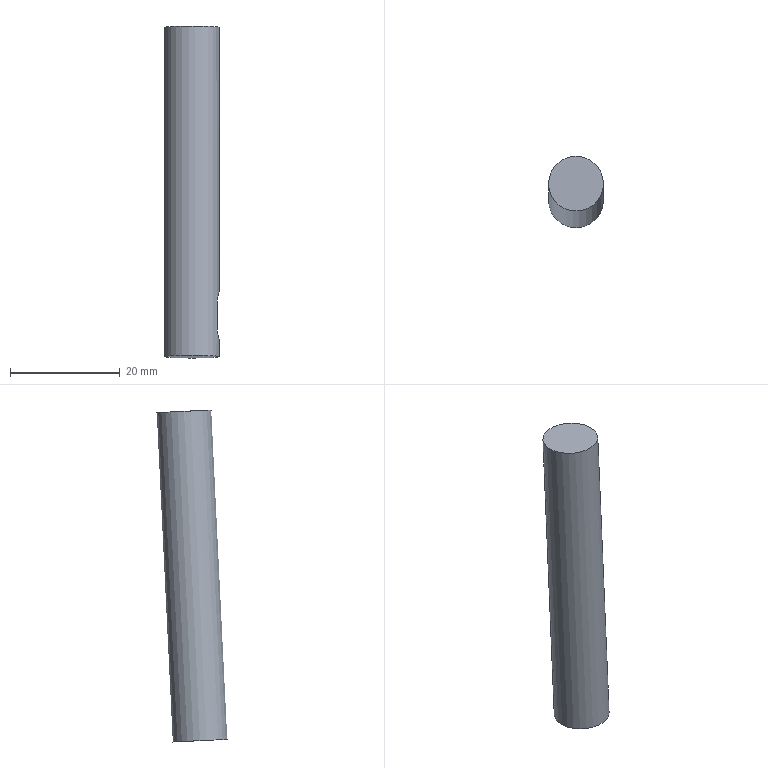Component | NX | CCJ-022 | 1 solid | 8 faces | box 10 x 12.91 x 60.42 mm | volume 4658 mm3 | plane 5 | cylinder 3 | commonest cylinder face diameters 4 x2 10 x1
STEP:
#1=CARTESIAN_POINT('',(0.,0.,0.));
#2=DIRECTION('',(0.,0.,1.));
#3=DIRECTION('',(1.,0.,0.));
#4=AXIS2_PLACEMENT_3D('',#1,#2,#3);
#5=CARTESIAN_POINT('',(30.,442.597,164.469));
#6=VERTEX_POINT('',#5);
#7=CARTESIAN_POINT('',(25.,442.597,164.469));
#8=DIRECTION('',(0.,0.04861,0.9988));
#9=DIRECTION('',(1.,0.,0.));
#10=AXIS2_PLACEMENT_3D('',#7,#8,#9);
#11=CIRCLE('',#10,5.);
#12=CARTESIAN_POINT('',(25.,445.514,224.398));
#13=DIRECTION('',(0.,-0.04861,-0.9988));
#14=DIRECTION('',(-1.,0.,0.));
#15=AXIS2_PLACEMENT_3D('',#12,#13,#14);
#16=CYLINDRICAL_SURFACE('',#15,5.);
#17=CARTESIAN_POINT('',(9.425,60.));
#18=DIRECTION('',(-1.,0.));
#19=VECTOR('',#18,1.);
#20=LINE('',#17,#19);
#21=(GEOMETRIC_REPRESENTATION_CONTEXT(2)PARAMETRIC_REPRESENTATION_CONTEXT()REPRESENTATION_CONTEXT('',''));
#22=DEFINITIONAL_REPRESENTATION('',(#20),#21);
#23=PCURVE('',#16,#22);
#24=CARTESIAN_POINT('',(25.,442.597,164.469));
#25=DIRECTION('',(0.,0.04861,0.9988));
#26=DIRECTION('',(1.,0.,0.));
#27=AXIS2_PLACEMENT_3D('',#24,#25,#26);
#28=PLANE('',#27);
#29=CARTESIAN_POINT('',(0.,0.));
#30=DIRECTION('',(1.,0.));
#31=AXIS2_PLACEMENT_2D('',#29,#30);
#32=CIRCLE('',#31,5.);
#33=(GEOMETRIC_REPRESENTATION_CONTEXT(2)PARAMETRIC_REPRESENTATION_CONTEXT()REPRESENTATION_CONTEXT('',''));
#34=DEFINITIONAL_REPRESENTATION('',(#32),#33);
#35=PCURVE('',#28,#34);
#36=SURFACE_CURVE('',#11,(#23,#35),.PCURVE_S1.);
#37=EDGE_CURVE('',#6,#6,#36,.T.);
#38=ORIENTED_EDGE('',*,*,#37,.T.);
#39=CARTESIAN_POINT('',(30.,442.743,167.466));
#40=VERTEX_POINT('',#39);
#41=CARTESIAN_POINT('',(30.,442.743,167.466));
#42=CARTESIAN_POINT('',(30.,442.597,164.469));
#43=B_SPLINE_CURVE_WITH_KNOTS('',1,(#41,#42),.UNSPECIFIED.,.F.,.F.,(2,2),(57.,60.),.PIECEWISE_BEZIER_KNOTS.);
#44=CARTESIAN_POINT('',(3.142,0.));
#45=DIRECTION('',(0.,1.));
#46=VECTOR('',#45,1.);
#47=LINE('',#44,#46);
#48=(GEOMETRIC_REPRESENTATION_CONTEXT(2)PARAMETRIC_REPRESENTATION_CONTEXT()REPRESENTATION_CONTEXT('',''));
#49=DEFINITIONAL_REPRESENTATION('',(#47),#48);
#50=PCURVE('',#16,#49);
#51=CARTESIAN_POINT('',(9.425,0.));
#52=DIRECTION('',(0.,1.));
#53=VECTOR('',#52,1.);
#54=LINE('',#51,#53);
#55=(GEOMETRIC_REPRESENTATION_CONTEXT(2)PARAMETRIC_REPRESENTATION_CONTEXT()REPRESENTATION_CONTEXT('',''));
#56=DEFINITIONAL_REPRESENTATION('',(#54),#55);
#57=PCURVE('',#16,#56);
#58=SEAM_CURVE('',#43,(#50,#57),.PCURVE_S1.);
#59=EDGE_CURVE('',#40,#6,#58,.T.);
#60=ORIENTED_EDGE('',*,*,#59,.F.);
#61=CARTESIAN_POINT('',(29.583,440.843,169.56));
#62=VERTEX_POINT('',#61);
#63=CARTESIAN_POINT('',(29.583,440.843,169.56));
#64=CARTESIAN_POINT('',(29.583,440.832,169.347));
#65=CARTESIAN_POINT('',(29.598,440.857,169.129));
#66=CARTESIAN_POINT('',(29.626,440.914,168.925));
#67=CARTESIAN_POINT('',(29.653,440.971,168.721));
#68=CARTESIAN_POINT('',(29.692,441.061,168.526));
#69=CARTESIAN_POINT('',(29.735,441.177,168.352));
#70=CARTESIAN_POINT('',(29.779,441.299,168.169));
#71=CARTESIAN_POINT('',(29.828,441.453,168.005));
#72=CARTESIAN_POINT('',(29.87,441.629,167.872));
#73=CARTESIAN_POINT('',(29.914,441.811,167.733));
#74=CARTESIAN_POINT('',(29.952,442.021,167.624));
#75=CARTESIAN_POINT('',(29.975,442.243,167.554));
#76=CARTESIAN_POINT('',(29.996,442.453,167.489));
#77=CARTESIAN_POINT('',(30.004,442.679,167.457));
#78=CARTESIAN_POINT('',(29.998,442.901,167.464));
#79=CARTESIAN_POINT('',(29.991,443.11,167.47));
#80=CARTESIAN_POINT('',(29.971,443.32,167.51));
#81=CARTESIAN_POINT('',(29.941,443.515,167.58));
#82=CARTESIAN_POINT('',(29.911,443.713,167.651));
#83=CARTESIAN_POINT('',(29.871,443.9,167.754));
#84=CARTESIAN_POINT('',(29.828,444.065,167.882));
#85=CARTESIAN_POINT('',(29.783,444.24,168.018));
#86=CARTESIAN_POINT('',(29.734,444.395,168.185));
#87=CARTESIAN_POINT('',(29.692,444.516,168.371));
#88=CARTESIAN_POINT('',(29.65,444.641,168.563));
#89=CARTESIAN_POINT('',(29.615,444.735,168.781));
#90=CARTESIAN_POINT('',(29.597,444.788,169.007));
#91=CARTESIAN_POINT('',(29.587,444.815,169.124));
#92=CARTESIAN_POINT('',(29.583,444.832,169.245));
#93=CARTESIAN_POINT('',(29.583,444.838,169.366));
#94=B_SPLINE_CURVE_WITH_KNOTS('',3,(#63,#64,#65,#66,#67,#68,#69,#70,#71,#72,#73,#74,#75,#76,#77,#78,#79,#80,#81,#82,#83,#84,#85,#86,#87,#88,#89,#90,#91,#92,#93),.UNSPECIFIED.,.F.,.F.,(4,3,3,3,3,3,3,3,3,3,4),(0.,0.1015,0.2026,0.309,0.4198,0.5251,0.6244,0.7251,0.8326,0.9432,1.),.UNSPECIFIED.);
#95=CARTESIAN_POINT('',(3.553,55.));
#96=CARTESIAN_POINT('',(3.553,55.048));
#97=CARTESIAN_POINT('',(3.552,55.144));
#98=CARTESIAN_POINT('',(3.549,55.287));
#99=CARTESIAN_POINT('',(3.543,55.43));
#100=CARTESIAN_POINT('',(3.536,55.569));
#101=CARTESIAN_POINT('',(3.526,55.704));
#102=CARTESIAN_POINT('',(3.514,55.836));
#103=CARTESIAN_POINT('',(3.5,55.963));
#104=CARTESIAN_POINT('',(3.485,56.085));
#105=CARTESIAN_POINT('',(3.468,56.201));
#106=CARTESIAN_POINT('',(3.449,56.311));
#107=CARTESIAN_POINT('',(3.429,56.415));
#108=CARTESIAN_POINT('',(3.407,56.511));
#109=CARTESIAN_POINT('',(3.384,56.6));
#110=CARTESIAN_POINT('',(3.361,56.681));
#111=CARTESIAN_POINT('',(3.336,56.754));
#112=CARTESIAN_POINT('',(3.31,56.818));
#113=CARTESIAN_POINT('',(3.283,56.873));
#114=CARTESIAN_POINT('',(3.256,56.919));
#115=CARTESIAN_POINT('',(3.228,56.955));
#116=CARTESIAN_POINT('',(3.2,56.98));
#117=CARTESIAN_POINT('',(3.171,56.996));
#118=CARTESIAN_POINT('',(3.142,57.002));
#119=CARTESIAN_POINT('',(3.113,56.997));
#120=CARTESIAN_POINT('',(3.084,56.981));
#121=CARTESIAN_POINT('',(3.056,56.955));
#122=CARTESIAN_POINT('',(3.028,56.92));
#123=CARTESIAN_POINT('',(3.,56.874));
#124=CARTESIAN_POINT('',(2.974,56.819));
#125=CARTESIAN_POINT('',(2.948,56.755));
#126=CARTESIAN_POINT('',(2.923,56.682));
#127=CARTESIAN_POINT('',(2.899,56.601));
#128=CARTESIAN_POINT('',(2.876,56.512));
#129=CARTESIAN_POINT('',(2.855,56.416));
#130=CARTESIAN_POINT('',(2.835,56.312));
#131=CARTESIAN_POINT('',(2.816,56.202));
#132=CARTESIAN_POINT('',(2.799,56.086));
#133=CARTESIAN_POINT('',(2.783,55.965));
#134=CARTESIAN_POINT('',(2.77,55.838));
#135=CARTESIAN_POINT('',(2.758,55.706));
#136=CARTESIAN_POINT('',(2.748,55.57));
#137=CARTESIAN_POINT('',(2.74,55.432));
#138=CARTESIAN_POINT('',(2.734,55.29));
#139=CARTESIAN_POINT('',(2.731,55.145));
#140=CARTESIAN_POINT('',(2.73,55.048));
#141=CARTESIAN_POINT('',(2.73,55.));
#142=B_SPLINE_CURVE_WITH_KNOTS('',3,(#95,#96,#97,#98,#99,#100,#101,#102,#103,#104,#105,#106,#107,#108,#109,#110,#111,#112,#113,#114,#115,#116,#117,#118,#119,#120,#121,#122,#123,#124,#125,#126,#127,#128,#129,#130,#131,#132,#133,#134,#135,#136,#137,#138,#139,#140,#141),.UNSPECIFIED.,.F.,.F.,(4,1,1,1,1,1,1,1,1,1,1,1,1,1,1,1,1,1,1,1,1,1,1,1,1,1,1,1,1,1,1,1,1,1,1,1,1,1,1,1,1,1,1,1,4),(0.,0.02273,0.04545,0.06818,0.09091,0.1136,0.1364,0.1591,0.1818,0.2045,0.2273,0.25,0.2727,0.2955,0.3182,0.3409,0.3636,0.3864,0.4091,0.4318,0.4545,0.4773,0.5,0.5227,0.5455,0.5682,0.5909,0.6136,0.6364,0.6591,0.6818,0.7045,0.7273,0.75,0.7727,0.7955,0.8182,0.8409,0.8636,0.8864,0.9091,0.9318,0.9545,0.9773,1.),.QUASI_UNIFORM_KNOTS.);
#143=(GEOMETRIC_REPRESENTATION_CONTEXT(2)PARAMETRIC_REPRESENTATION_CONTEXT()REPRESENTATION_CONTEXT('',''));
#144=DEFINITIONAL_REPRESENTATION('',(#142),#143);
#145=PCURVE('',#16,#144);
#146=CARTESIAN_POINT('',(40.,442.84,169.463));
#147=DIRECTION('',(-1.,0.,0.));
#148=DIRECTION('',(0.,0.04861,0.9988));
#149=AXIS2_PLACEMENT_3D('',#146,#147,#148);
#150=CYLINDRICAL_SURFACE('',#149,2.);
#151=CARTESIAN_POINT('',(4.712,10.417));
#152=CARTESIAN_POINT('',(3.142,10.));
#153=B_SPLINE_CURVE_WITH_KNOTS('',1,(#151,#152),.UNSPECIFIED.,.F.,.F.,(2,2),(0.,0.5002),.PIECEWISE_BEZIER_KNOTS.);
#154=(GEOMETRIC_REPRESENTATION_CONTEXT(2)PARAMETRIC_REPRESENTATION_CONTEXT()REPRESENTATION_CONTEXT('',''));
#155=DEFINITIONAL_REPRESENTATION('',(#153),#154);
#156=PCURVE('',#150,#155);
#157=SURFACE_CURVE('',#94,(#145,#156),.PCURVE_S1.);
#158=EDGE_CURVE('',#62,#40,#157,.T.);
#159=ORIENTED_EDGE('',*,*,#158,.F.);
#160=CARTESIAN_POINT('',(29.583,441.086,174.554));
#161=VERTEX_POINT('',#160);
#162=CARTESIAN_POINT('',(29.583,443.516,224.495));
#163=DIRECTION('',(0.,-0.04861,-0.9988));
#164=VECTOR('',#163,1.);
#165=LINE('',#162,#164);
#166=CARTESIAN_POINT('',(3.553,0.));
#167=DIRECTION('',(-0.,1.));
#168=VECTOR('',#167,1.);
#169=LINE('',#166,#168);
#170=(GEOMETRIC_REPRESENTATION_CONTEXT(2)PARAMETRIC_REPRESENTATION_CONTEXT()REPRESENTATION_CONTEXT('',''));
#171=DEFINITIONAL_REPRESENTATION('',(#169),#170);
#172=PCURVE('',#16,#171);
#173=CARTESIAN_POINT('',(40.,441.086,174.554));
#174=DIRECTION('',(0.,0.9988,-0.04861));
#175=DIRECTION('',(0.,0.04861,0.9988));
#176=AXIS2_PLACEMENT_3D('',#173,#174,#175);
#177=PLANE('',#176);
#178=CARTESIAN_POINT('',(50.,-10.417));
#179=DIRECTION('',(-1.,0.));
#180=VECTOR('',#179,1.);
#181=LINE('',#178,#180);
#182=(GEOMETRIC_REPRESENTATION_CONTEXT(2)PARAMETRIC_REPRESENTATION_CONTEXT()REPRESENTATION_CONTEXT('',''));
#183=DEFINITIONAL_REPRESENTATION('',(#181),#182);
#184=PCURVE('',#177,#183);
#185=SURFACE_CURVE('',#165,(#172,#184),.PCURVE_S1.);
#186=EDGE_CURVE('',#161,#62,#185,.T.);
#187=ORIENTED_EDGE('',*,*,#186,.F.);
#188=CARTESIAN_POINT('',(30.,443.181,176.455));
#189=VERTEX_POINT('',#188);
#190=CARTESIAN_POINT('',(29.583,445.081,174.36));
#191=CARTESIAN_POINT('',(29.583,445.091,174.573));
#192=CARTESIAN_POINT('',(29.598,445.067,174.791));
#193=CARTESIAN_POINT('',(29.626,445.01,174.995));
#194=CARTESIAN_POINT('',(29.653,444.953,175.199));
#195=CARTESIAN_POINT('',(29.692,444.862,175.394));
#196=CARTESIAN_POINT('',(29.735,444.746,175.568));
#197=CARTESIAN_POINT('',(29.779,444.624,175.751));
#198=CARTESIAN_POINT('',(29.828,444.47,175.915));
#199=CARTESIAN_POINT('',(29.87,444.295,176.048));
#200=CARTESIAN_POINT('',(29.914,444.113,176.187));
#201=CARTESIAN_POINT('',(29.952,443.902,176.296));
#202=CARTESIAN_POINT('',(29.975,443.681,176.366));
#203=CARTESIAN_POINT('',(29.996,443.471,176.432));
#204=CARTESIAN_POINT('',(30.004,443.244,176.463));
#205=CARTESIAN_POINT('',(29.998,443.023,176.456));
#206=CARTESIAN_POINT('',(29.991,442.814,176.45));
#207=CARTESIAN_POINT('',(29.971,442.604,176.41));
#208=CARTESIAN_POINT('',(29.941,442.409,176.34));
#209=CARTESIAN_POINT('',(29.911,442.211,176.269));
#210=CARTESIAN_POINT('',(29.871,442.023,176.166));
#211=CARTESIAN_POINT('',(29.828,441.859,176.038));
#212=CARTESIAN_POINT('',(29.783,441.683,175.902));
#213=CARTESIAN_POINT('',(29.734,441.529,175.735));
#214=CARTESIAN_POINT('',(29.692,441.408,175.549));
#215=CARTESIAN_POINT('',(29.65,441.283,175.357));
#216=CARTESIAN_POINT('',(29.615,441.189,175.139));
#217=CARTESIAN_POINT('',(29.597,441.136,174.913));
#218=CARTESIAN_POINT('',(29.587,441.109,174.796));
#219=CARTESIAN_POINT('',(29.583,441.092,174.675));
#220=CARTESIAN_POINT('',(29.583,441.086,174.554));
#221=B_SPLINE_CURVE_WITH_KNOTS('',3,(#190,#191,#192,#193,#194,#195,#196,#197,#198,#199,#200,#201,#202,#203,#204,#205,#206,#207,#208,#209,#210,#211,#212,#213,#214,#215,#216,#217,#218,#219,#220),.UNSPECIFIED.,.F.,.F.,(4,3,3,3,3,3,3,3,3,3,4),(0.,0.1015,0.2026,0.309,0.4198,0.5251,0.6244,0.7251,0.8326,0.9432,1.),.UNSPECIFIED.);
#222=CARTESIAN_POINT('',(2.73,50.));
#223=CARTESIAN_POINT('',(2.73,49.952));
#224=CARTESIAN_POINT('',(2.731,49.856));
#225=CARTESIAN_POINT('',(2.734,49.713));
#226=CARTESIAN_POINT('',(2.74,49.57));
#227=CARTESIAN_POINT('',(2.748,49.431));
#228=CARTESIAN_POINT('',(2.757,49.296));
#229=CARTESIAN_POINT('',(2.769,49.164));
#230=CARTESIAN_POINT('',(2.783,49.037));
#231=CARTESIAN_POINT('',(2.799,48.915));
#232=CARTESIAN_POINT('',(2.816,48.799));
#233=CARTESIAN_POINT('',(2.834,48.689));
#234=CARTESIAN_POINT('',(2.855,48.585));
#235=CARTESIAN_POINT('',(2.876,48.489));
#236=CARTESIAN_POINT('',(2.899,48.4));
#237=CARTESIAN_POINT('',(2.923,48.319));
#238=CARTESIAN_POINT('',(2.947,48.246));
#239=CARTESIAN_POINT('',(2.973,48.182));
#240=CARTESIAN_POINT('',(3.,48.127));
#241=CARTESIAN_POINT('',(3.027,48.081));
#242=CARTESIAN_POINT('',(3.055,48.045));
#243=CARTESIAN_POINT('',(3.084,48.02));
#244=CARTESIAN_POINT('',(3.112,48.004));
#245=CARTESIAN_POINT('',(3.141,47.998));
#246=CARTESIAN_POINT('',(3.17,48.003));
#247=CARTESIAN_POINT('',(3.199,48.019));
#248=CARTESIAN_POINT('',(3.227,48.045));
#249=CARTESIAN_POINT('',(3.255,48.08));
#250=CARTESIAN_POINT('',(3.283,48.126));
#251=CARTESIAN_POINT('',(3.309,48.181));
#252=CARTESIAN_POINT('',(3.335,48.245));
#253=CARTESIAN_POINT('',(3.36,48.318));
#254=CARTESIAN_POINT('',(3.384,48.399));
#255=CARTESIAN_POINT('',(3.407,48.488));
#256=CARTESIAN_POINT('',(3.428,48.584));
#257=CARTESIAN_POINT('',(3.449,48.688));
#258=CARTESIAN_POINT('',(3.467,48.798));
#259=CARTESIAN_POINT('',(3.485,48.914));
#260=CARTESIAN_POINT('',(3.5,49.035));
#261=CARTESIAN_POINT('',(3.514,49.162));
#262=CARTESIAN_POINT('',(3.525,49.294));
#263=CARTESIAN_POINT('',(3.535,49.43));
#264=CARTESIAN_POINT('',(3.543,49.568));
#265=CARTESIAN_POINT('',(3.549,49.71));
#266=CARTESIAN_POINT('',(3.552,49.855));
#267=CARTESIAN_POINT('',(3.553,49.952));
#268=CARTESIAN_POINT('',(3.553,50.));
#269=B_SPLINE_CURVE_WITH_KNOTS('',3,(#222,#223,#224,#225,#226,#227,#228,#229,#230,#231,#232,#233,#234,#235,#236,#237,#238,#239,#240,#241,#242,#243,#244,#245,#246,#247,#248,#249,#250,#251,#252,#253,#254,#255,#256,#257,#258,#259,#260,#261,#262,#263,#264,#265,#266,#267,#268),.UNSPECIFIED.,.F.,.F.,(4,1,1,1,1,1,1,1,1,1,1,1,1,1,1,1,1,1,1,1,1,1,1,1,1,1,1,1,1,1,1,1,1,1,1,1,1,1,1,1,1,1,1,1,4),(0.,0.02273,0.04545,0.06818,0.09091,0.1136,0.1364,0.1591,0.1818,0.2045,0.2273,0.25,0.2727,0.2955,0.3182,0.3409,0.3636,0.3864,0.4091,0.4318,0.4545,0.4773,0.5,0.5227,0.5455,0.5682,0.5909,0.6136,0.6364,0.6591,0.6818,0.7045,0.7273,0.75,0.7727,0.7955,0.8182,0.8409,0.8636,0.8864,0.9091,0.9318,0.9545,0.9773,1.),.QUASI_UNIFORM_KNOTS.);
#270=(GEOMETRIC_REPRESENTATION_CONTEXT(2)PARAMETRIC_REPRESENTATION_CONTEXT()REPRESENTATION_CONTEXT('',''));
#271=DEFINITIONAL_REPRESENTATION('',(#269),#270);
#272=PCURVE('',#16,#271);
#273=CARTESIAN_POINT('',(40.,443.083,174.457));
#274=DIRECTION('',(-1.,0.,0.));
#275=DIRECTION('',(0.,0.04861,0.9988));
#276=AXIS2_PLACEMENT_3D('',#273,#274,#275);
#277=CYLINDRICAL_SURFACE('',#276,2.);
#278=CARTESIAN_POINT('',(6.283,10.));
#279=CARTESIAN_POINT('',(4.712,10.417));
#280=B_SPLINE_CURVE_WITH_KNOTS('',1,(#278,#279),.UNSPECIFIED.,.F.,.F.,(2,2),(0.5002,1.),.PIECEWISE_BEZIER_KNOTS.);
#281=(GEOMETRIC_REPRESENTATION_CONTEXT(2)PARAMETRIC_REPRESENTATION_CONTEXT()REPRESENTATION_CONTEXT('',''));
#282=DEFINITIONAL_REPRESENTATION('',(#280),#281);
#283=PCURVE('',#277,#282);
#284=SURFACE_CURVE('',#221,(#272,#283),.PCURVE_S1.);
#285=EDGE_CURVE('',#189,#161,#284,.T.);
#286=ORIENTED_EDGE('',*,*,#285,.F.);
#287=CARTESIAN_POINT('',(30.,445.514,224.398));
#288=VERTEX_POINT('',#287);
#289=CARTESIAN_POINT('',(30.,445.514,224.398));
#290=CARTESIAN_POINT('',(30.,443.181,176.455));
#291=B_SPLINE_CURVE_WITH_KNOTS('',1,(#289,#290),.UNSPECIFIED.,.F.,.F.,(2,2),(0.,48.),.PIECEWISE_BEZIER_KNOTS.);
#292=CARTESIAN_POINT('',(3.142,0.));
#293=DIRECTION('',(0.,1.));
#294=VECTOR('',#293,1.);
#295=LINE('',#292,#294);
#296=(GEOMETRIC_REPRESENTATION_CONTEXT(2)PARAMETRIC_REPRESENTATION_CONTEXT()REPRESENTATION_CONTEXT('',''));
#297=DEFINITIONAL_REPRESENTATION('',(#295),#296);
#298=PCURVE('',#16,#297);
#299=CARTESIAN_POINT('',(9.425,0.));
#300=DIRECTION('',(0.,1.));
#301=VECTOR('',#300,1.);
#302=LINE('',#299,#301);
#303=(GEOMETRIC_REPRESENTATION_CONTEXT(2)PARAMETRIC_REPRESENTATION_CONTEXT()REPRESENTATION_CONTEXT('',''));
#304=DEFINITIONAL_REPRESENTATION('',(#302),#303);
#305=PCURVE('',#16,#304);
#306=SEAM_CURVE('',#291,(#298,#305),.PCURVE_S1.);
#307=EDGE_CURVE('',#288,#189,#306,.T.);
#308=ORIENTED_EDGE('',*,*,#307,.F.);
#309=CARTESIAN_POINT('',(25.,445.514,224.398));
#310=DIRECTION('',(0.,0.04861,0.9988));
#311=DIRECTION('',(1.,0.,0.));
#312=AXIS2_PLACEMENT_3D('',#309,#310,#311);
#313=CIRCLE('',#312,5.);
#314=CARTESIAN_POINT('',(9.425,0.));
#315=DIRECTION('',(-1.,0.));
#316=VECTOR('',#315,1.);
#317=LINE('',#314,#316);
#318=(GEOMETRIC_REPRESENTATION_CONTEXT(2)PARAMETRIC_REPRESENTATION_CONTEXT()REPRESENTATION_CONTEXT('',''));
#319=DEFINITIONAL_REPRESENTATION('',(#317),#318);
#320=PCURVE('',#16,#319);
#321=CARTESIAN_POINT('',(25.,445.514,224.398));
#322=DIRECTION('',(0.,0.04861,0.9988));
#323=DIRECTION('',(1.,0.,0.));
#324=AXIS2_PLACEMENT_3D('',#321,#322,#323);
#325=PLANE('',#324);
#326=CARTESIAN_POINT('',(0.,0.));
#327=DIRECTION('',(1.,0.));
#328=AXIS2_PLACEMENT_2D('',#326,#327);
#329=CIRCLE('',#328,5.);
#330=(GEOMETRIC_REPRESENTATION_CONTEXT(2)PARAMETRIC_REPRESENTATION_CONTEXT()REPRESENTATION_CONTEXT('',''));
#331=DEFINITIONAL_REPRESENTATION('',(#329),#330);
#332=PCURVE('',#325,#331);
#333=SURFACE_CURVE('',#313,(#320,#332),.PCURVE_S1.);
#334=EDGE_CURVE('',#288,#288,#333,.T.);
#335=ORIENTED_EDGE('',*,*,#334,.F.);
#336=ORIENTED_EDGE('',*,*,#307,.T.);
#337=CARTESIAN_POINT('',(29.583,445.081,174.36));
#338=VERTEX_POINT('',#337);
#339=CARTESIAN_POINT('',(29.583,445.081,174.36));
#340=CARTESIAN_POINT('',(29.583,445.091,174.573));
#341=CARTESIAN_POINT('',(29.598,445.067,174.791));
#342=CARTESIAN_POINT('',(29.626,445.01,174.995));
#343=CARTESIAN_POINT('',(29.653,444.953,175.199));
#344=CARTESIAN_POINT('',(29.692,444.862,175.394));
#345=CARTESIAN_POINT('',(29.735,444.746,175.568));
#346=CARTESIAN_POINT('',(29.779,444.624,175.751));
#347=CARTESIAN_POINT('',(29.828,444.47,175.915));
#348=CARTESIAN_POINT('',(29.87,444.295,176.048));
#349=CARTESIAN_POINT('',(29.914,444.113,176.187));
#350=CARTESIAN_POINT('',(29.952,443.902,176.296));
#351=CARTESIAN_POINT('',(29.975,443.681,176.366));
#352=CARTESIAN_POINT('',(29.996,443.471,176.432));
#353=CARTESIAN_POINT('',(30.004,443.244,176.463));
#354=CARTESIAN_POINT('',(29.998,443.023,176.456));
#355=CARTESIAN_POINT('',(29.991,442.814,176.45));
#356=CARTESIAN_POINT('',(29.971,442.604,176.41));
#357=CARTESIAN_POINT('',(29.941,442.409,176.34));
#358=CARTESIAN_POINT('',(29.911,442.211,176.269));
#359=CARTESIAN_POINT('',(29.871,442.023,176.166));
#360=CARTESIAN_POINT('',(29.828,441.859,176.038));
#361=CARTESIAN_POINT('',(29.783,441.683,175.902));
#362=CARTESIAN_POINT('',(29.734,441.529,175.735));
#363=CARTESIAN_POINT('',(29.692,441.408,175.549));
#364=CARTESIAN_POINT('',(29.65,441.283,175.357));
#365=CARTESIAN_POINT('',(29.615,441.189,175.139));
#366=CARTESIAN_POINT('',(29.597,441.136,174.913));
#367=CARTESIAN_POINT('',(29.587,441.109,174.796));
#368=CARTESIAN_POINT('',(29.583,441.092,174.675));
#369=CARTESIAN_POINT('',(29.583,441.086,174.554));
#370=B_SPLINE_CURVE_WITH_KNOTS('',3,(#339,#340,#341,#342,#343,#344,#345,#346,#347,#348,#349,#350,#351,#352,#353,#354,#355,#356,#357,#358,#359,#360,#361,#362,#363,#364,#365,#366,#367,#368,#369),.UNSPECIFIED.,.F.,.F.,(4,3,3,3,3,3,3,3,3,3,4),(0.,0.1015,0.2026,0.309,0.4198,0.5251,0.6244,0.7251,0.8326,0.9432,1.),.UNSPECIFIED.);
#371=CARTESIAN_POINT('',(9.013,50.));
#372=CARTESIAN_POINT('',(9.013,49.952));
#373=CARTESIAN_POINT('',(9.014,49.856));
#374=CARTESIAN_POINT('',(9.017,49.713));
#375=CARTESIAN_POINT('',(9.023,49.57));
#376=CARTESIAN_POINT('',(9.031,49.431));
#377=CARTESIAN_POINT('',(9.041,49.296));
#378=CARTESIAN_POINT('',(9.052,49.164));
#379=CARTESIAN_POINT('',(9.066,49.037));
#380=CARTESIAN_POINT('',(9.082,48.915));
#381=CARTESIAN_POINT('',(9.099,48.799));
#382=CARTESIAN_POINT('',(9.117,48.689));
#383=CARTESIAN_POINT('',(9.138,48.585));
#384=CARTESIAN_POINT('',(9.159,48.489));
#385=CARTESIAN_POINT('',(9.182,48.4));
#386=CARTESIAN_POINT('',(9.206,48.319));
#387=CARTESIAN_POINT('',(9.231,48.246));
#388=CARTESIAN_POINT('',(9.257,48.182));
#389=CARTESIAN_POINT('',(9.283,48.127));
#390=CARTESIAN_POINT('',(9.311,48.081));
#391=CARTESIAN_POINT('',(9.338,48.045));
#392=CARTESIAN_POINT('',(9.367,48.02));
#393=CARTESIAN_POINT('',(9.396,48.004));
#394=CARTESIAN_POINT('',(9.425,47.998));
#395=CARTESIAN_POINT('',(9.453,48.003));
#396=CARTESIAN_POINT('',(9.482,48.019));
#397=CARTESIAN_POINT('',(9.51,48.045));
#398=CARTESIAN_POINT('',(9.538,48.08));
#399=CARTESIAN_POINT('',(9.566,48.126));
#400=CARTESIAN_POINT('',(9.592,48.181));
#401=CARTESIAN_POINT('',(9.618,48.245));
#402=CARTESIAN_POINT('',(9.643,48.318));
#403=CARTESIAN_POINT('',(9.667,48.399));
#404=CARTESIAN_POINT('',(9.69,48.488));
#405=CARTESIAN_POINT('',(9.712,48.584));
#406=CARTESIAN_POINT('',(9.732,48.688));
#407=CARTESIAN_POINT('',(9.751,48.798));
#408=CARTESIAN_POINT('',(9.768,48.914));
#409=CARTESIAN_POINT('',(9.783,49.035));
#410=CARTESIAN_POINT('',(9.797,49.162));
#411=CARTESIAN_POINT('',(9.809,49.294));
#412=CARTESIAN_POINT('',(9.819,49.43));
#413=CARTESIAN_POINT('',(9.826,49.568));
#414=CARTESIAN_POINT('',(9.832,49.71));
#415=CARTESIAN_POINT('',(9.836,49.855));
#416=CARTESIAN_POINT('',(9.836,49.952));
#417=CARTESIAN_POINT('',(9.836,50.));
#418=B_SPLINE_CURVE_WITH_KNOTS('',3,(#371,#372,#373,#374,#375,#376,#377,#378,#379,#380,#381,#382,#383,#384,#385,#386,#387,#388,#389,#390,#391,#392,#393,#394,#395,#396,#397,#398,#399,#400,#401,#402,#403,#404,#405,#406,#407,#408,#409,#410,#411,#412,#413,#414,#415,#416,#417),.UNSPECIFIED.,.F.,.F.,(4,1,1,1,1,1,1,1,1,1,1,1,1,1,1,1,1,1,1,1,1,1,1,1,1,1,1,1,1,1,1,1,1,1,1,1,1,1,1,1,1,1,1,1,4),(0.,0.02273,0.04545,0.06818,0.09091,0.1136,0.1364,0.1591,0.1818,0.2045,0.2273,0.25,0.2727,0.2955,0.3182,0.3409,0.3636,0.3864,0.4091,0.4318,0.4545,0.4773,0.5,0.5227,0.5455,0.5682,0.5909,0.6136,0.6364,0.6591,0.6818,0.7045,0.7273,0.75,0.7727,0.7955,0.8182,0.8409,0.8636,0.8864,0.9091,0.9318,0.9545,0.9773,1.),.QUASI_UNIFORM_KNOTS.);
#419=(GEOMETRIC_REPRESENTATION_CONTEXT(2)PARAMETRIC_REPRESENTATION_CONTEXT()REPRESENTATION_CONTEXT('',''));
#420=DEFINITIONAL_REPRESENTATION('',(#418),#419);
#421=PCURVE('',#16,#420);
#422=CARTESIAN_POINT('',(7.854,10.417));
#423=CARTESIAN_POINT('',(6.283,10.));
#424=B_SPLINE_CURVE_WITH_KNOTS('',1,(#422,#423),.UNSPECIFIED.,.F.,.F.,(2,2),(0.,0.5002),.PIECEWISE_BEZIER_KNOTS.);
#425=(GEOMETRIC_REPRESENTATION_CONTEXT(2)PARAMETRIC_REPRESENTATION_CONTEXT()REPRESENTATION_CONTEXT('',''));
#426=DEFINITIONAL_REPRESENTATION('',(#424),#425);
#427=PCURVE('',#277,#426);
#428=SURFACE_CURVE('',#370,(#421,#427),.PCURVE_S1.);
#429=EDGE_CURVE('',#338,#189,#428,.T.);
#430=ORIENTED_EDGE('',*,*,#429,.F.);
#431=CARTESIAN_POINT('',(29.583,444.838,169.366));
#432=VERTEX_POINT('',#431);
#433=CARTESIAN_POINT('',(29.583,447.512,224.301));
#434=DIRECTION('',(0.,0.04861,0.9988));
#435=VECTOR('',#434,1.);
#436=LINE('',#433,#435);
#437=CARTESIAN_POINT('',(9.013,-0.));
#438=DIRECTION('',(0.,-1.));
#439=VECTOR('',#438,1.);
#440=LINE('',#437,#439);
#441=(GEOMETRIC_REPRESENTATION_CONTEXT(2)PARAMETRIC_REPRESENTATION_CONTEXT()REPRESENTATION_CONTEXT('',''));
#442=DEFINITIONAL_REPRESENTATION('',(#440),#441);
#443=PCURVE('',#16,#442);
#444=CARTESIAN_POINT('',(40.,444.838,169.366));
#445=DIRECTION('',(0.,-0.9988,0.04861));
#446=DIRECTION('',(0.,-0.04861,-0.9988));
#447=AXIS2_PLACEMENT_3D('',#444,#445,#446);
#448=PLANE('',#447);
#449=CARTESIAN_POINT('',(-55.,-10.417));
#450=DIRECTION('',(-1.,0.));
#451=VECTOR('',#450,1.);
#452=LINE('',#449,#451);
#453=(GEOMETRIC_REPRESENTATION_CONTEXT(2)PARAMETRIC_REPRESENTATION_CONTEXT()REPRESENTATION_CONTEXT('',''));
#454=DEFINITIONAL_REPRESENTATION('',(#452),#453);
#455=PCURVE('',#448,#454);
#456=SURFACE_CURVE('',#436,(#443,#455),.PCURVE_S1.);
#457=EDGE_CURVE('',#432,#338,#456,.T.);
#458=ORIENTED_EDGE('',*,*,#457,.F.);
#459=CARTESIAN_POINT('',(29.583,440.843,169.56));
#460=CARTESIAN_POINT('',(29.583,440.832,169.347));
#461=CARTESIAN_POINT('',(29.598,440.857,169.129));
#462=CARTESIAN_POINT('',(29.626,440.914,168.925));
#463=CARTESIAN_POINT('',(29.653,440.971,168.721));
#464=CARTESIAN_POINT('',(29.692,441.061,168.526));
#465=CARTESIAN_POINT('',(29.735,441.177,168.352));
#466=CARTESIAN_POINT('',(29.779,441.299,168.169));
#467=CARTESIAN_POINT('',(29.828,441.453,168.005));
#468=CARTESIAN_POINT('',(29.87,441.629,167.872));
#469=CARTESIAN_POINT('',(29.914,441.811,167.733));
#470=CARTESIAN_POINT('',(29.952,442.021,167.624));
#471=CARTESIAN_POINT('',(29.975,442.243,167.554));
#472=CARTESIAN_POINT('',(29.996,442.453,167.489));
#473=CARTESIAN_POINT('',(30.004,442.679,167.457));
#474=CARTESIAN_POINT('',(29.998,442.901,167.464));
#475=CARTESIAN_POINT('',(29.991,443.11,167.47));
#476=CARTESIAN_POINT('',(29.971,443.32,167.51));
#477=CARTESIAN_POINT('',(29.941,443.515,167.58));
#478=CARTESIAN_POINT('',(29.911,443.713,167.651));
#479=CARTESIAN_POINT('',(29.871,443.9,167.754));
#480=CARTESIAN_POINT('',(29.828,444.065,167.882));
#481=CARTESIAN_POINT('',(29.783,444.24,168.018));
#482=CARTESIAN_POINT('',(29.734,444.395,168.185));
#483=CARTESIAN_POINT('',(29.692,444.516,168.371));
#484=CARTESIAN_POINT('',(29.65,444.641,168.563));
#485=CARTESIAN_POINT('',(29.615,444.735,168.781));
#486=CARTESIAN_POINT('',(29.597,444.788,169.007));
#487=CARTESIAN_POINT('',(29.587,444.815,169.124));
#488=CARTESIAN_POINT('',(29.583,444.832,169.245));
#489=CARTESIAN_POINT('',(29.583,444.838,169.366));
#490=B_SPLINE_CURVE_WITH_KNOTS('',3,(#459,#460,#461,#462,#463,#464,#465,#466,#467,#468,#469,#470,#471,#472,#473,#474,#475,#476,#477,#478,#479,#480,#481,#482,#483,#484,#485,#486,#487,#488,#489),.UNSPECIFIED.,.F.,.F.,(4,3,3,3,3,3,3,3,3,3,4),(0.,0.1015,0.2026,0.309,0.4198,0.5251,0.6244,0.7251,0.8326,0.9432,1.),.UNSPECIFIED.);
#491=CARTESIAN_POINT('',(9.836,55.));
#492=CARTESIAN_POINT('',(9.836,55.048));
#493=CARTESIAN_POINT('',(9.836,55.144));
#494=CARTESIAN_POINT('',(9.832,55.287));
#495=CARTESIAN_POINT('',(9.826,55.43));
#496=CARTESIAN_POINT('',(9.819,55.569));
#497=CARTESIAN_POINT('',(9.809,55.704));
#498=CARTESIAN_POINT('',(9.797,55.836));
#499=CARTESIAN_POINT('',(9.783,55.963));
#500=CARTESIAN_POINT('',(9.768,56.085));
#501=CARTESIAN_POINT('',(9.751,56.201));
#502=CARTESIAN_POINT('',(9.732,56.311));
#503=CARTESIAN_POINT('',(9.712,56.415));
#504=CARTESIAN_POINT('',(9.69,56.511));
#505=CARTESIAN_POINT('',(9.668,56.6));
#506=CARTESIAN_POINT('',(9.644,56.681));
#507=CARTESIAN_POINT('',(9.619,56.754));
#508=CARTESIAN_POINT('',(9.593,56.818));
#509=CARTESIAN_POINT('',(9.566,56.873));
#510=CARTESIAN_POINT('',(9.539,56.919));
#511=CARTESIAN_POINT('',(9.511,56.955));
#512=CARTESIAN_POINT('',(9.483,56.98));
#513=CARTESIAN_POINT('',(9.454,56.996));
#514=CARTESIAN_POINT('',(9.425,57.002));
#515=CARTESIAN_POINT('',(9.396,56.997));
#516=CARTESIAN_POINT('',(9.368,56.981));
#517=CARTESIAN_POINT('',(9.339,56.955));
#518=CARTESIAN_POINT('',(9.311,56.92));
#519=CARTESIAN_POINT('',(9.284,56.874));
#520=CARTESIAN_POINT('',(9.257,56.819));
#521=CARTESIAN_POINT('',(9.231,56.755));
#522=CARTESIAN_POINT('',(9.206,56.682));
#523=CARTESIAN_POINT('',(9.182,56.601));
#524=CARTESIAN_POINT('',(9.159,56.512));
#525=CARTESIAN_POINT('',(9.138,56.416));
#526=CARTESIAN_POINT('',(9.118,56.312));
#527=CARTESIAN_POINT('',(9.099,56.202));
#528=CARTESIAN_POINT('',(9.082,56.086));
#529=CARTESIAN_POINT('',(9.066,55.965));
#530=CARTESIAN_POINT('',(9.053,55.838));
#531=CARTESIAN_POINT('',(9.041,55.706));
#532=CARTESIAN_POINT('',(9.031,55.57));
#533=CARTESIAN_POINT('',(9.023,55.432));
#534=CARTESIAN_POINT('',(9.017,55.29));
#535=CARTESIAN_POINT('',(9.014,55.145));
#536=CARTESIAN_POINT('',(9.013,55.048));
#537=CARTESIAN_POINT('',(9.013,55.));
#538=B_SPLINE_CURVE_WITH_KNOTS('',3,(#491,#492,#493,#494,#495,#496,#497,#498,#499,#500,#501,#502,#503,#504,#505,#506,#507,#508,#509,#510,#511,#512,#513,#514,#515,#516,#517,#518,#519,#520,#521,#522,#523,#524,#525,#526,#527,#528,#529,#530,#531,#532,#533,#534,#535,#536,#537),.UNSPECIFIED.,.F.,.F.,(4,1,1,1,1,1,1,1,1,1,1,1,1,1,1,1,1,1,1,1,1,1,1,1,1,1,1,1,1,1,1,1,1,1,1,1,1,1,1,1,1,1,1,1,4),(0.,0.02273,0.04545,0.06818,0.09091,0.1136,0.1364,0.1591,0.1818,0.2045,0.2273,0.25,0.2727,0.2955,0.3182,0.3409,0.3636,0.3864,0.4091,0.4318,0.4545,0.4773,0.5,0.5227,0.5455,0.5682,0.5909,0.6136,0.6364,0.6591,0.6818,0.7045,0.7273,0.75,0.7727,0.7955,0.8182,0.8409,0.8636,0.8864,0.9091,0.9318,0.9545,0.9773,1.),.QUASI_UNIFORM_KNOTS.);
#539=(GEOMETRIC_REPRESENTATION_CONTEXT(2)PARAMETRIC_REPRESENTATION_CONTEXT()REPRESENTATION_CONTEXT('',''));
#540=DEFINITIONAL_REPRESENTATION('',(#538),#539);
#541=PCURVE('',#16,#540);
#542=CARTESIAN_POINT('',(3.142,10.));
#543=CARTESIAN_POINT('',(1.571,10.417));
#544=B_SPLINE_CURVE_WITH_KNOTS('',1,(#542,#543),.UNSPECIFIED.,.F.,.F.,(2,2),(0.5002,1.),.PIECEWISE_BEZIER_KNOTS.);
#545=(GEOMETRIC_REPRESENTATION_CONTEXT(2)PARAMETRIC_REPRESENTATION_CONTEXT()REPRESENTATION_CONTEXT('',''));
#546=DEFINITIONAL_REPRESENTATION('',(#544),#545);
#547=PCURVE('',#150,#546);
#548=SURFACE_CURVE('',#490,(#541,#547),.PCURVE_S1.);
#549=EDGE_CURVE('',#40,#432,#548,.T.);
#550=ORIENTED_EDGE('',*,*,#549,.F.);
#551=ORIENTED_EDGE('',*,*,#59,.T.);
#552=EDGE_LOOP('',(#38,#60,#159,#187,#286,#308,#335,#336,#430,#458,#550,#551));
#553=FACE_BOUND('',#552,.T.);
#554=ADVANCED_FACE('',(#553),#16,.T.);
#555=ORIENTED_EDGE('',*,*,#334,.T.);
#556=EDGE_LOOP('',(#555));
#557=FACE_BOUND('',#556,.T.);
#558=ADVANCED_FACE('',(#557),#325,.T.);
#559=ORIENTED_EDGE('',*,*,#37,.F.);
#560=EDGE_LOOP('',(#559));
#561=FACE_BOUND('',#560,.T.);
#562=ADVANCED_FACE('',(#561),#28,.F.);
#563=ORIENTED_EDGE('',*,*,#186,.T.);
#564=CARTESIAN_POINT('',(28.2,440.843,169.56));
#565=VERTEX_POINT('',#564);
#566=CARTESIAN_POINT('',(40.,440.843,169.56));
#567=DIRECTION('',(1.,0.,0.));
#568=VECTOR('',#567,1.);
#569=LINE('',#566,#568);
#570=CARTESIAN_POINT('',(-5.,0.));
#571=DIRECTION('',(0.,1.));
#572=VECTOR('',#571,1.);
#573=LINE('',#570,#572);
#574=(GEOMETRIC_REPRESENTATION_CONTEXT(2)PARAMETRIC_REPRESENTATION_CONTEXT()REPRESENTATION_CONTEXT('',''));
#575=DEFINITIONAL_REPRESENTATION('',(#573),#574);
#576=PCURVE('',#177,#575);
#577=CARTESIAN_POINT('',(4.712,0.));
#578=DIRECTION('',(0.,-1.));
#579=VECTOR('',#578,1.);
#580=LINE('',#577,#579);
#581=(GEOMETRIC_REPRESENTATION_CONTEXT(2)PARAMETRIC_REPRESENTATION_CONTEXT()REPRESENTATION_CONTEXT('',''));
#582=DEFINITIONAL_REPRESENTATION('',(#580),#581);
#583=PCURVE('',#150,#582);
#584=SURFACE_CURVE('',#569,(#576,#583),.PCURVE_S1.);
#585=EDGE_CURVE('',#565,#62,#584,.T.);
#586=ORIENTED_EDGE('',*,*,#585,.F.);
#587=CARTESIAN_POINT('',(28.2,441.086,174.554));
#588=VERTEX_POINT('',#587);
#589=CARTESIAN_POINT('',(28.2,441.086,174.554));
#590=DIRECTION('',(0.,0.04861,0.9988));
#591=VECTOR('',#590,1.);
#592=LINE('',#589,#591);
#593=CARTESIAN_POINT('',(0.,-11.8));
#594=DIRECTION('',(1.,0.));
#595=VECTOR('',#594,1.);
#596=LINE('',#593,#595);
#597=(GEOMETRIC_REPRESENTATION_CONTEXT(2)PARAMETRIC_REPRESENTATION_CONTEXT()REPRESENTATION_CONTEXT('',''));
#598=DEFINITIONAL_REPRESENTATION('',(#596),#597);
#599=PCURVE('',#177,#598);
#600=CARTESIAN_POINT('',(28.2,442.84,169.463));
#601=DIRECTION('',(1.,0.,0.));
#602=DIRECTION('',(0.,-0.04861,-0.9988));
#603=AXIS2_PLACEMENT_3D('',#600,#601,#602);
#604=PLANE('',#603);
#605=CARTESIAN_POINT('',(-5.,-2.));
#606=DIRECTION('',(-1.,0.));
#607=VECTOR('',#606,1.);
#608=LINE('',#605,#607);
#609=(GEOMETRIC_REPRESENTATION_CONTEXT(2)PARAMETRIC_REPRESENTATION_CONTEXT()REPRESENTATION_CONTEXT('',''));
#610=DEFINITIONAL_REPRESENTATION('',(#608),#609);
#611=PCURVE('',#604,#610);
#612=SURFACE_CURVE('',#592,(#599,#611),.PCURVE_S1.);
#613=EDGE_CURVE('',#565,#588,#612,.T.);
#614=ORIENTED_EDGE('',*,*,#613,.T.);
#615=CARTESIAN_POINT('',(40.,441.086,174.554));
#616=DIRECTION('',(1.,0.,0.));
#617=VECTOR('',#616,1.);
#618=LINE('',#615,#617);
#619=CARTESIAN_POINT('',(0.,0.));
#620=DIRECTION('',(0.,1.));
#621=VECTOR('',#620,1.);
#622=LINE('',#619,#621);
#623=(GEOMETRIC_REPRESENTATION_CONTEXT(2)PARAMETRIC_REPRESENTATION_CONTEXT()REPRESENTATION_CONTEXT('',''));
#624=DEFINITIONAL_REPRESENTATION('',(#622),#623);
#625=PCURVE('',#177,#624);
#626=CARTESIAN_POINT('',(4.712,0.));
#627=DIRECTION('',(0.,-1.));
#628=VECTOR('',#627,1.);
#629=LINE('',#626,#628);
#630=(GEOMETRIC_REPRESENTATION_CONTEXT(2)PARAMETRIC_REPRESENTATION_CONTEXT()REPRESENTATION_CONTEXT('',''));
#631=DEFINITIONAL_REPRESENTATION('',(#629),#630);
#632=PCURVE('',#277,#631);
#633=SURFACE_CURVE('',#618,(#625,#632),.PCURVE_S1.);
#634=EDGE_CURVE('',#588,#161,#633,.T.);
#635=ORIENTED_EDGE('',*,*,#634,.T.);
#636=EDGE_LOOP('',(#563,#586,#614,#635));
#637=FACE_BOUND('',#636,.T.);
#638=ADVANCED_FACE('',(#637),#177,.T.);
#639=ORIENTED_EDGE('',*,*,#585,.F.);
#640=CARTESIAN_POINT('',(28.2,444.838,169.366));
#641=VERTEX_POINT('',#640);
#642=CARTESIAN_POINT('',(28.2,442.84,169.463));
#643=DIRECTION('',(-1.,0.,0.));
#644=DIRECTION('',(0.,0.9988,-0.04861));
#645=AXIS2_PLACEMENT_3D('',#642,#643,#644);
#646=CIRCLE('',#645,2.);
#647=CARTESIAN_POINT('',(1.571,11.8));
#648=DIRECTION('',(1.,0.));
#649=VECTOR('',#648,1.);
#650=LINE('',#647,#649);
#651=(GEOMETRIC_REPRESENTATION_CONTEXT(2)PARAMETRIC_REPRESENTATION_CONTEXT()REPRESENTATION_CONTEXT('',''));
#652=DEFINITIONAL_REPRESENTATION('',(#650),#651);
#653=PCURVE('',#150,#652);
#654=CARTESIAN_POINT('',(0.,2.));
#655=CARTESIAN_POINT('',(3.464,2.));
#656=CARTESIAN_POINT('',(1.732,-1.));
#657=CARTESIAN_POINT('',(-0.,-4.));
#658=CARTESIAN_POINT('',(-1.732,-1.));
#659=CARTESIAN_POINT('',(-3.464,2.));
#660=CARTESIAN_POINT('',(0.,2.));
#661=(BOUNDED_CURVE()B_SPLINE_CURVE(2,(#654,#655,#656,#657,#658,#659,#660),.UNSPECIFIED.,.T.,.F.)B_SPLINE_CURVE_WITH_KNOTS((1,2,2,2,2,1),(-2.094,0.,2.094,4.189,6.283,8.378),.UNSPECIFIED.)CURVE()GEOMETRIC_REPRESENTATION_ITEM()RATIONAL_B_SPLINE_CURVE((1.,0.5,1.,0.5,1.,0.5,1.))REPRESENTATION_ITEM(''));
#662=(GEOMETRIC_REPRESENTATION_CONTEXT(2)PARAMETRIC_REPRESENTATION_CONTEXT()REPRESENTATION_CONTEXT('',''));
#663=DEFINITIONAL_REPRESENTATION('',(#661),#662);
#664=PCURVE('',#604,#663);
#665=SURFACE_CURVE('',#646,(#653,#664),.PCURVE_S1.);
#666=EDGE_CURVE('',#641,#565,#665,.T.);
#667=ORIENTED_EDGE('',*,*,#666,.F.);
#668=CARTESIAN_POINT('',(40.,444.838,169.366));
#669=DIRECTION('',(1.,0.,0.));
#670=VECTOR('',#669,1.);
#671=LINE('',#668,#670);
#672=CARTESIAN_POINT('',(1.571,0.));
#673=DIRECTION('',(0.,-1.));
#674=VECTOR('',#673,1.);
#675=LINE('',#672,#674);
#676=(GEOMETRIC_REPRESENTATION_CONTEXT(2)PARAMETRIC_REPRESENTATION_CONTEXT()REPRESENTATION_CONTEXT('',''));
#677=DEFINITIONAL_REPRESENTATION('',(#675),#676);
#678=PCURVE('',#150,#677);
#679=CARTESIAN_POINT('',(0.,0.));
#680=DIRECTION('',(0.,1.));
#681=VECTOR('',#680,1.);
#682=LINE('',#679,#681);
#683=(GEOMETRIC_REPRESENTATION_CONTEXT(2)PARAMETRIC_REPRESENTATION_CONTEXT()REPRESENTATION_CONTEXT('',''));
#684=DEFINITIONAL_REPRESENTATION('',(#682),#683);
#685=PCURVE('',#448,#684);
#686=SURFACE_CURVE('',#671,(#678,#685),.PCURVE_S1.);
#687=EDGE_CURVE('',#641,#432,#686,.T.);
#688=ORIENTED_EDGE('',*,*,#687,.T.);
#689=ORIENTED_EDGE('',*,*,#549,.F.);
#690=ORIENTED_EDGE('',*,*,#158,.F.);
#691=EDGE_LOOP('',(#639,#667,#688,#689,#690));
#692=FACE_BOUND('',#691,.F.);
#693=ADVANCED_FACE('',(#692),#150,.F.);
#694=ORIENTED_EDGE('',*,*,#457,.T.);
#695=CARTESIAN_POINT('',(28.2,445.081,174.36));
#696=VERTEX_POINT('',#695);
#697=CARTESIAN_POINT('',(40.,445.081,174.36));
#698=DIRECTION('',(1.,0.,0.));
#699=VECTOR('',#698,1.);
#700=LINE('',#697,#699);
#701=CARTESIAN_POINT('',(-5.,0.));
#702=DIRECTION('',(0.,1.));
#703=VECTOR('',#702,1.);
#704=LINE('',#701,#703);
#705=(GEOMETRIC_REPRESENTATION_CONTEXT(2)PARAMETRIC_REPRESENTATION_CONTEXT()REPRESENTATION_CONTEXT('',''));
#706=DEFINITIONAL_REPRESENTATION('',(#704),#705);
#707=PCURVE('',#448,#706);
#708=CARTESIAN_POINT('',(7.854,0.));
#709=DIRECTION('',(0.,-1.));
#710=VECTOR('',#709,1.);
#711=LINE('',#708,#710);
#712=(GEOMETRIC_REPRESENTATION_CONTEXT(2)PARAMETRIC_REPRESENTATION_CONTEXT()REPRESENTATION_CONTEXT('',''));
#713=DEFINITIONAL_REPRESENTATION('',(#711),#712);
#714=PCURVE('',#277,#713);
#715=SURFACE_CURVE('',#700,(#707,#714),.PCURVE_S1.);
#716=EDGE_CURVE('',#696,#338,#715,.T.);
#717=ORIENTED_EDGE('',*,*,#716,.F.);
#718=CARTESIAN_POINT('',(28.2,444.838,169.366));
#719=DIRECTION('',(0.,-0.04861,-0.9988));
#720=VECTOR('',#719,1.);
#721=LINE('',#718,#720);
#722=CARTESIAN_POINT('',(0.,-11.8));
#723=DIRECTION('',(1.,0.));
#724=VECTOR('',#723,1.);
#725=LINE('',#722,#724);
#726=(GEOMETRIC_REPRESENTATION_CONTEXT(2)PARAMETRIC_REPRESENTATION_CONTEXT()REPRESENTATION_CONTEXT('',''));
#727=DEFINITIONAL_REPRESENTATION('',(#725),#726);
#728=PCURVE('',#448,#727);
#729=CARTESIAN_POINT('',(-0.,2.));
#730=DIRECTION('',(1.,0.));
#731=VECTOR('',#730,1.);
#732=LINE('',#729,#731);
#733=(GEOMETRIC_REPRESENTATION_CONTEXT(2)PARAMETRIC_REPRESENTATION_CONTEXT()REPRESENTATION_CONTEXT('',''));
#734=DEFINITIONAL_REPRESENTATION('',(#732),#733);
#735=PCURVE('',#604,#734);
#736=SURFACE_CURVE('',#721,(#728,#735),.PCURVE_S1.);
#737=EDGE_CURVE('',#696,#641,#736,.T.);
#738=ORIENTED_EDGE('',*,*,#737,.T.);
#739=ORIENTED_EDGE('',*,*,#687,.T.);
#740=EDGE_LOOP('',(#694,#717,#738,#739));
#741=FACE_BOUND('',#740,.T.);
#742=ADVANCED_FACE('',(#741),#448,.T.);
#743=ORIENTED_EDGE('',*,*,#716,.F.);
#744=CARTESIAN_POINT('',(28.2,443.083,174.457));
#745=DIRECTION('',(-1.,0.,0.));
#746=DIRECTION('',(0.,0.9988,-0.04861));
#747=AXIS2_PLACEMENT_3D('',#744,#745,#746);
#748=CIRCLE('',#747,2.);
#749=CARTESIAN_POINT('',(1.571,11.8));
#750=DIRECTION('',(1.,0.));
#751=VECTOR('',#750,1.);
#752=LINE('',#749,#751);
#753=(GEOMETRIC_REPRESENTATION_CONTEXT(2)PARAMETRIC_REPRESENTATION_CONTEXT()REPRESENTATION_CONTEXT('',''));
#754=DEFINITIONAL_REPRESENTATION('',(#752),#753);
#755=PCURVE('',#277,#754);
#756=CARTESIAN_POINT('',(-5.,2.));
#757=CARTESIAN_POINT('',(-1.536,2.));
#758=CARTESIAN_POINT('',(-3.268,-1.));
#759=CARTESIAN_POINT('',(-5.,-4.));
#760=CARTESIAN_POINT('',(-6.732,-1.));
#761=CARTESIAN_POINT('',(-8.464,2.));
#762=CARTESIAN_POINT('',(-5.,2.));
#763=(BOUNDED_CURVE()B_SPLINE_CURVE(2,(#756,#757,#758,#759,#760,#761,#762),.UNSPECIFIED.,.T.,.F.)B_SPLINE_CURVE_WITH_KNOTS((1,2,2,2,2,1),(-2.094,0.,2.094,4.189,6.283,8.378),.UNSPECIFIED.)CURVE()GEOMETRIC_REPRESENTATION_ITEM()RATIONAL_B_SPLINE_CURVE((1.,0.5,1.,0.5,1.,0.5,1.))REPRESENTATION_ITEM(''));
#764=(GEOMETRIC_REPRESENTATION_CONTEXT(2)PARAMETRIC_REPRESENTATION_CONTEXT()REPRESENTATION_CONTEXT('',''));
#765=DEFINITIONAL_REPRESENTATION('',(#763),#764);
#766=PCURVE('',#604,#765);
#767=SURFACE_CURVE('',#748,(#755,#766),.PCURVE_S1.);
#768=EDGE_CURVE('',#588,#696,#767,.T.);
#769=ORIENTED_EDGE('',*,*,#768,.F.);
#770=ORIENTED_EDGE('',*,*,#634,.T.);
#771=ORIENTED_EDGE('',*,*,#285,.F.);
#772=ORIENTED_EDGE('',*,*,#429,.F.);
#773=EDGE_LOOP('',(#743,#769,#770,#771,#772));
#774=FACE_BOUND('',#773,.F.);
#775=ADVANCED_FACE('',(#774),#277,.F.);
#776=ORIENTED_EDGE('',*,*,#613,.F.);
#777=ORIENTED_EDGE('',*,*,#666,.F.);
#778=ORIENTED_EDGE('',*,*,#737,.F.);
#779=ORIENTED_EDGE('',*,*,#768,.F.);
#780=EDGE_LOOP('',(#776,#777,#778,#779));
#781=FACE_BOUND('',#780,.T.);
#782=ADVANCED_FACE('',(#781),#604,.T.);
#783=CLOSED_SHELL('',(#554,#558,#562,#638,#693,#742,#775,#782));
#784=MANIFOLD_SOLID_BREP('',#783);
#785=(LENGTH_UNIT()NAMED_UNIT(*)SI_UNIT(.MILLI.,.METRE.));
#786=UNCERTAINTY_MEASURE_WITH_UNIT(LENGTH_MEASURE(0.02),#785,'','');
#787=(NAMED_UNIT(*)PLANE_ANGLE_UNIT()SI_UNIT($,.RADIAN.));
#788=(NAMED_UNIT(*)SI_UNIT($,.STERADIAN.)SOLID_ANGLE_UNIT());
#789=(GEOMETRIC_REPRESENTATION_CONTEXT(3)GLOBAL_UNCERTAINTY_ASSIGNED_CONTEXT((#786))GLOBAL_UNIT_ASSIGNED_CONTEXT((#785,#787,#788))REPRESENTATION_CONTEXT('',''));
#790=ADVANCED_BREP_SHAPE_REPRESENTATION('',(#4,#784),#789);